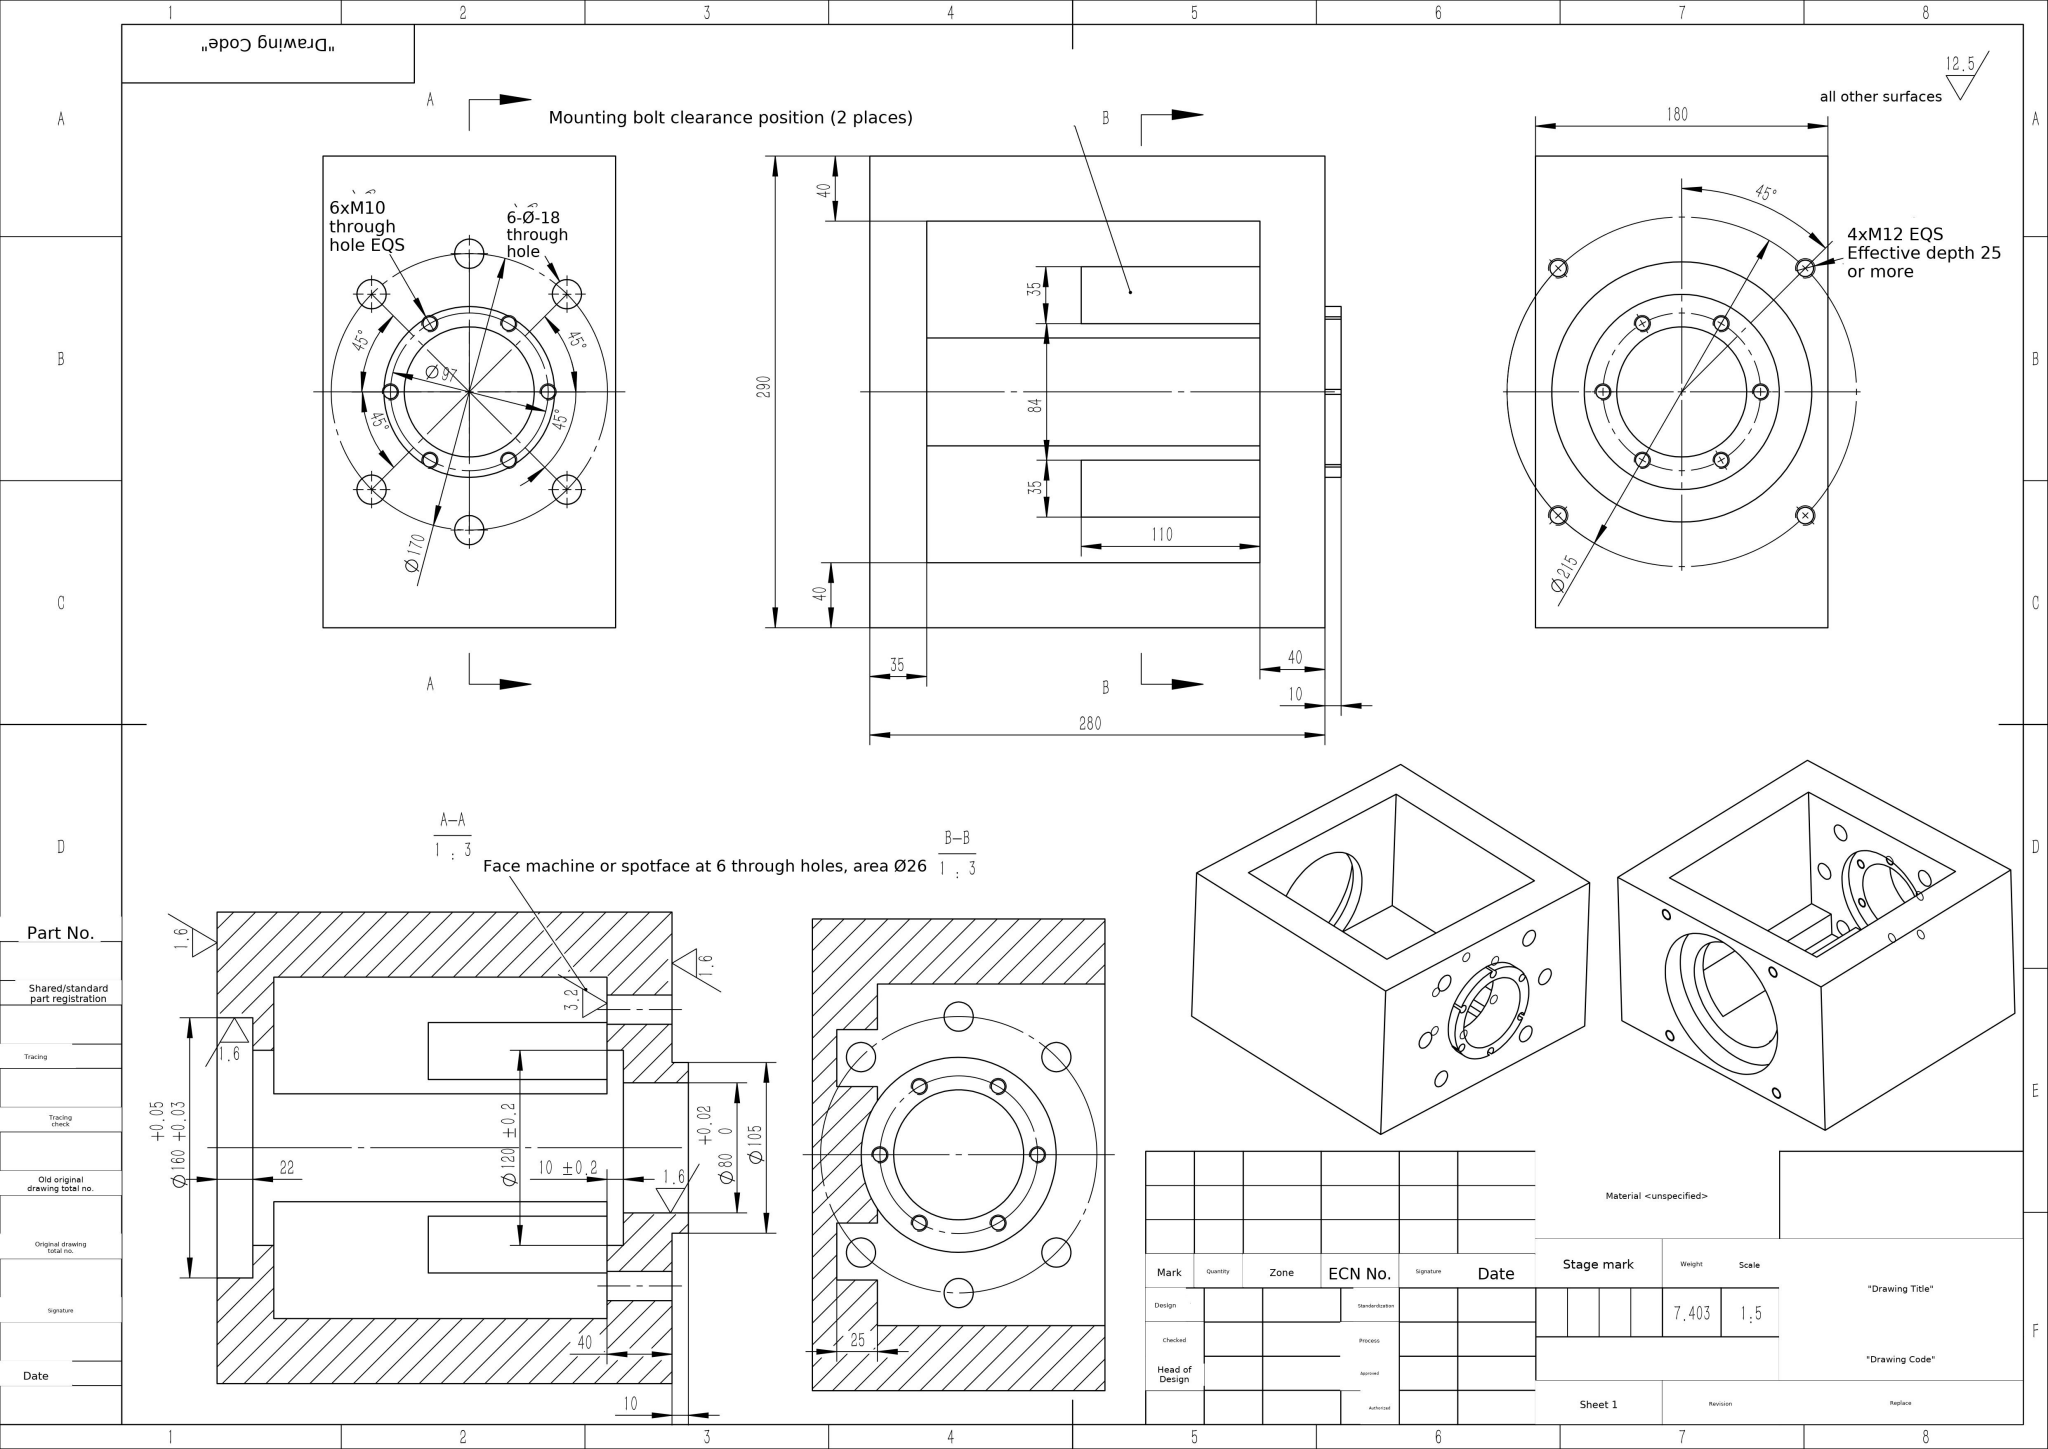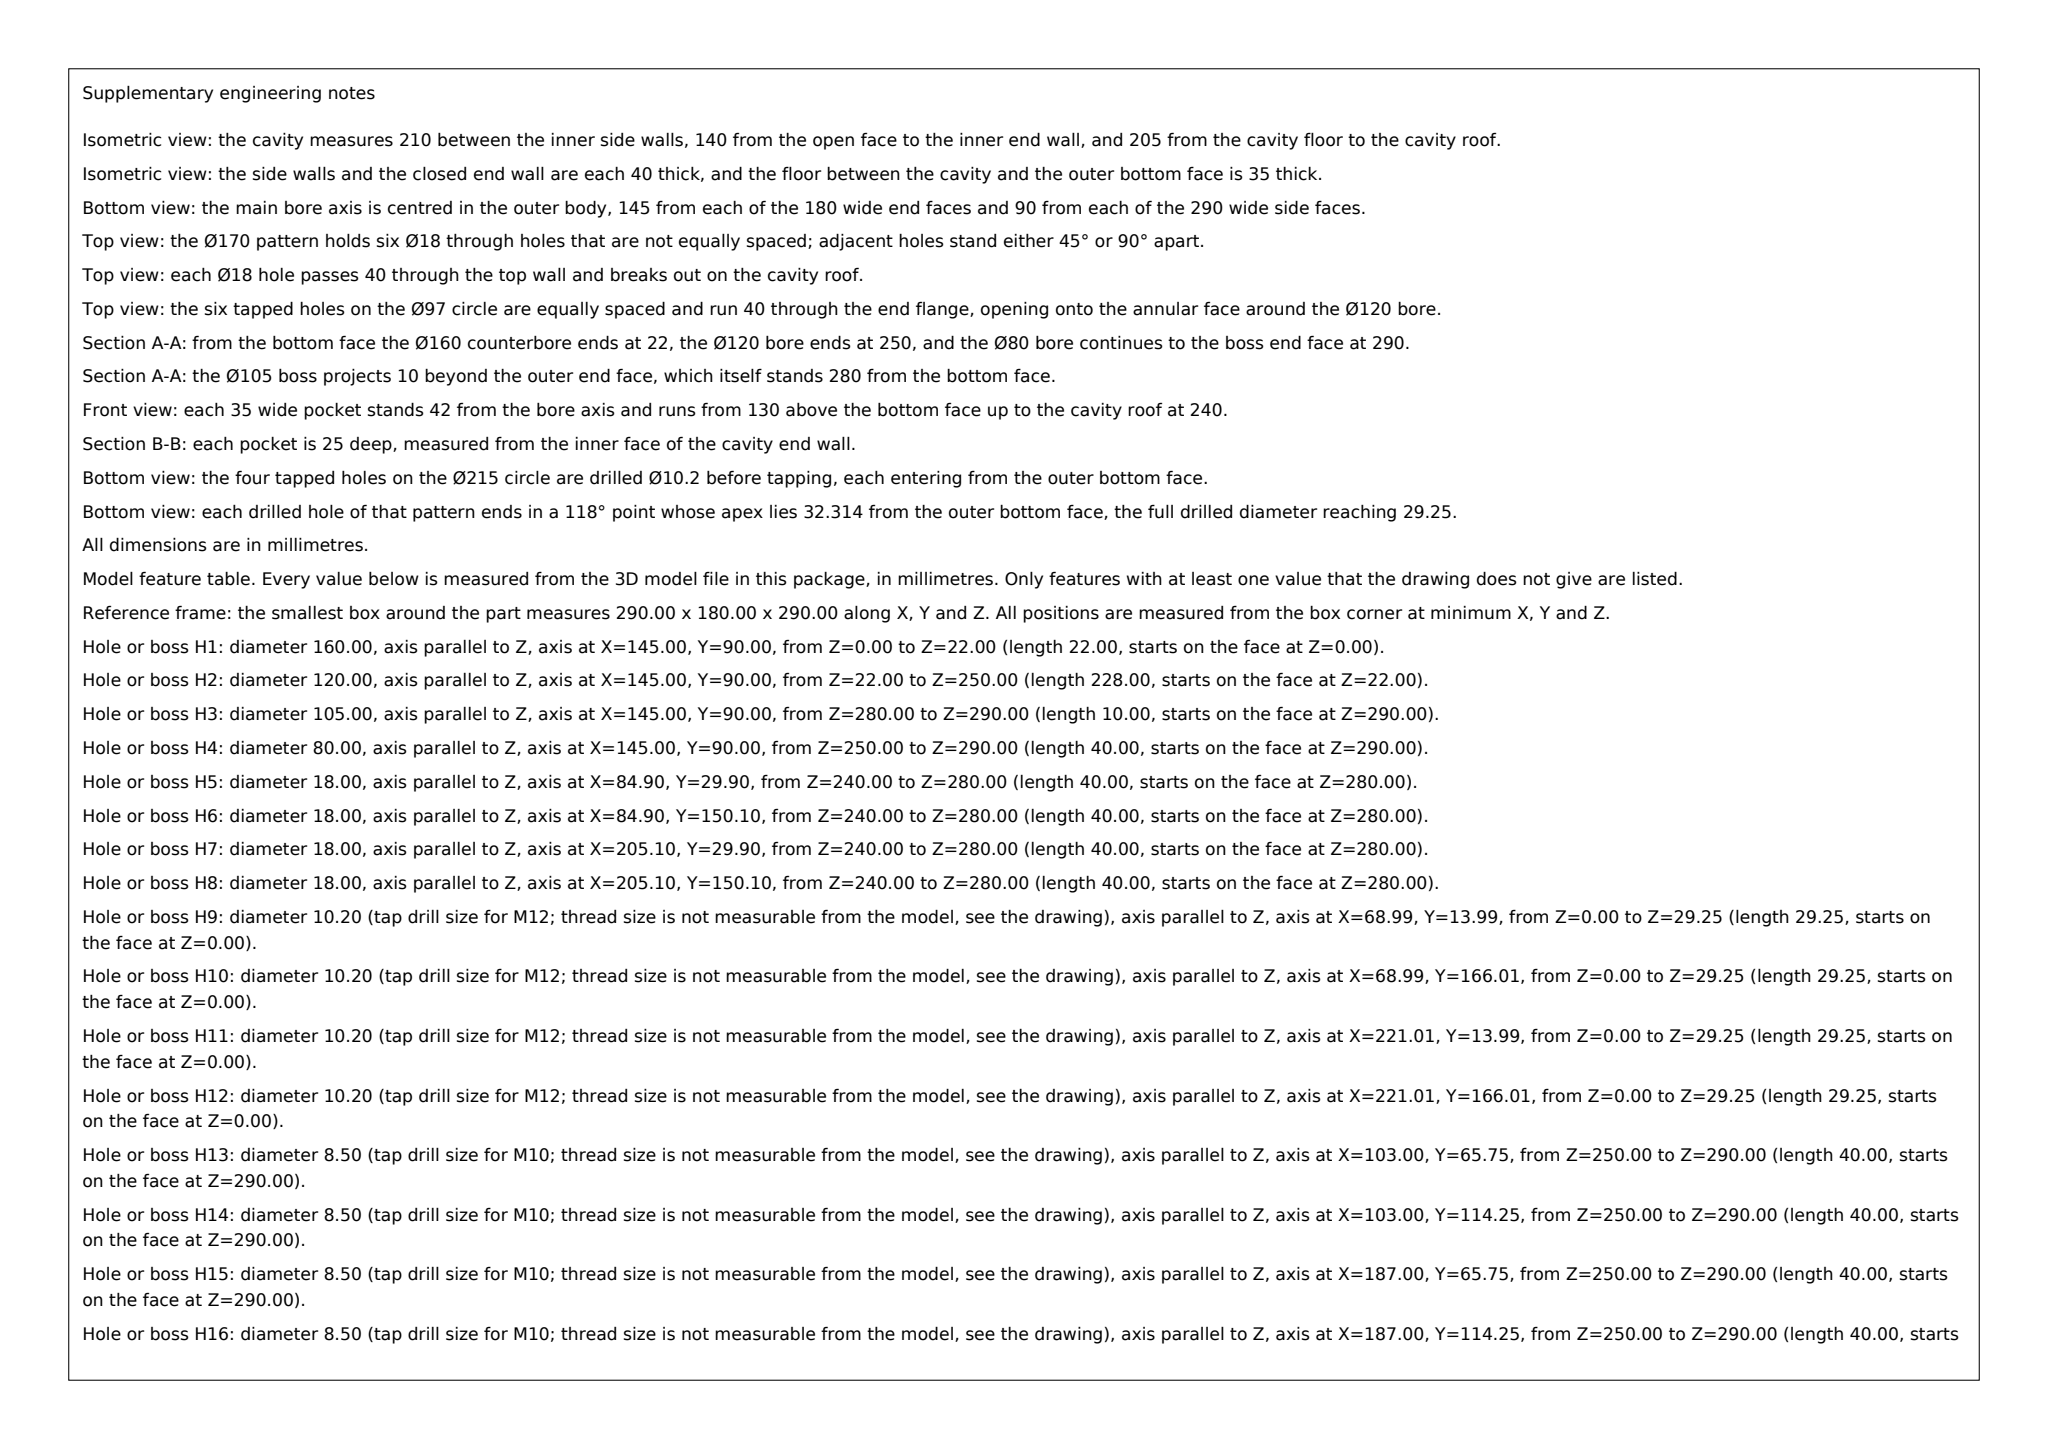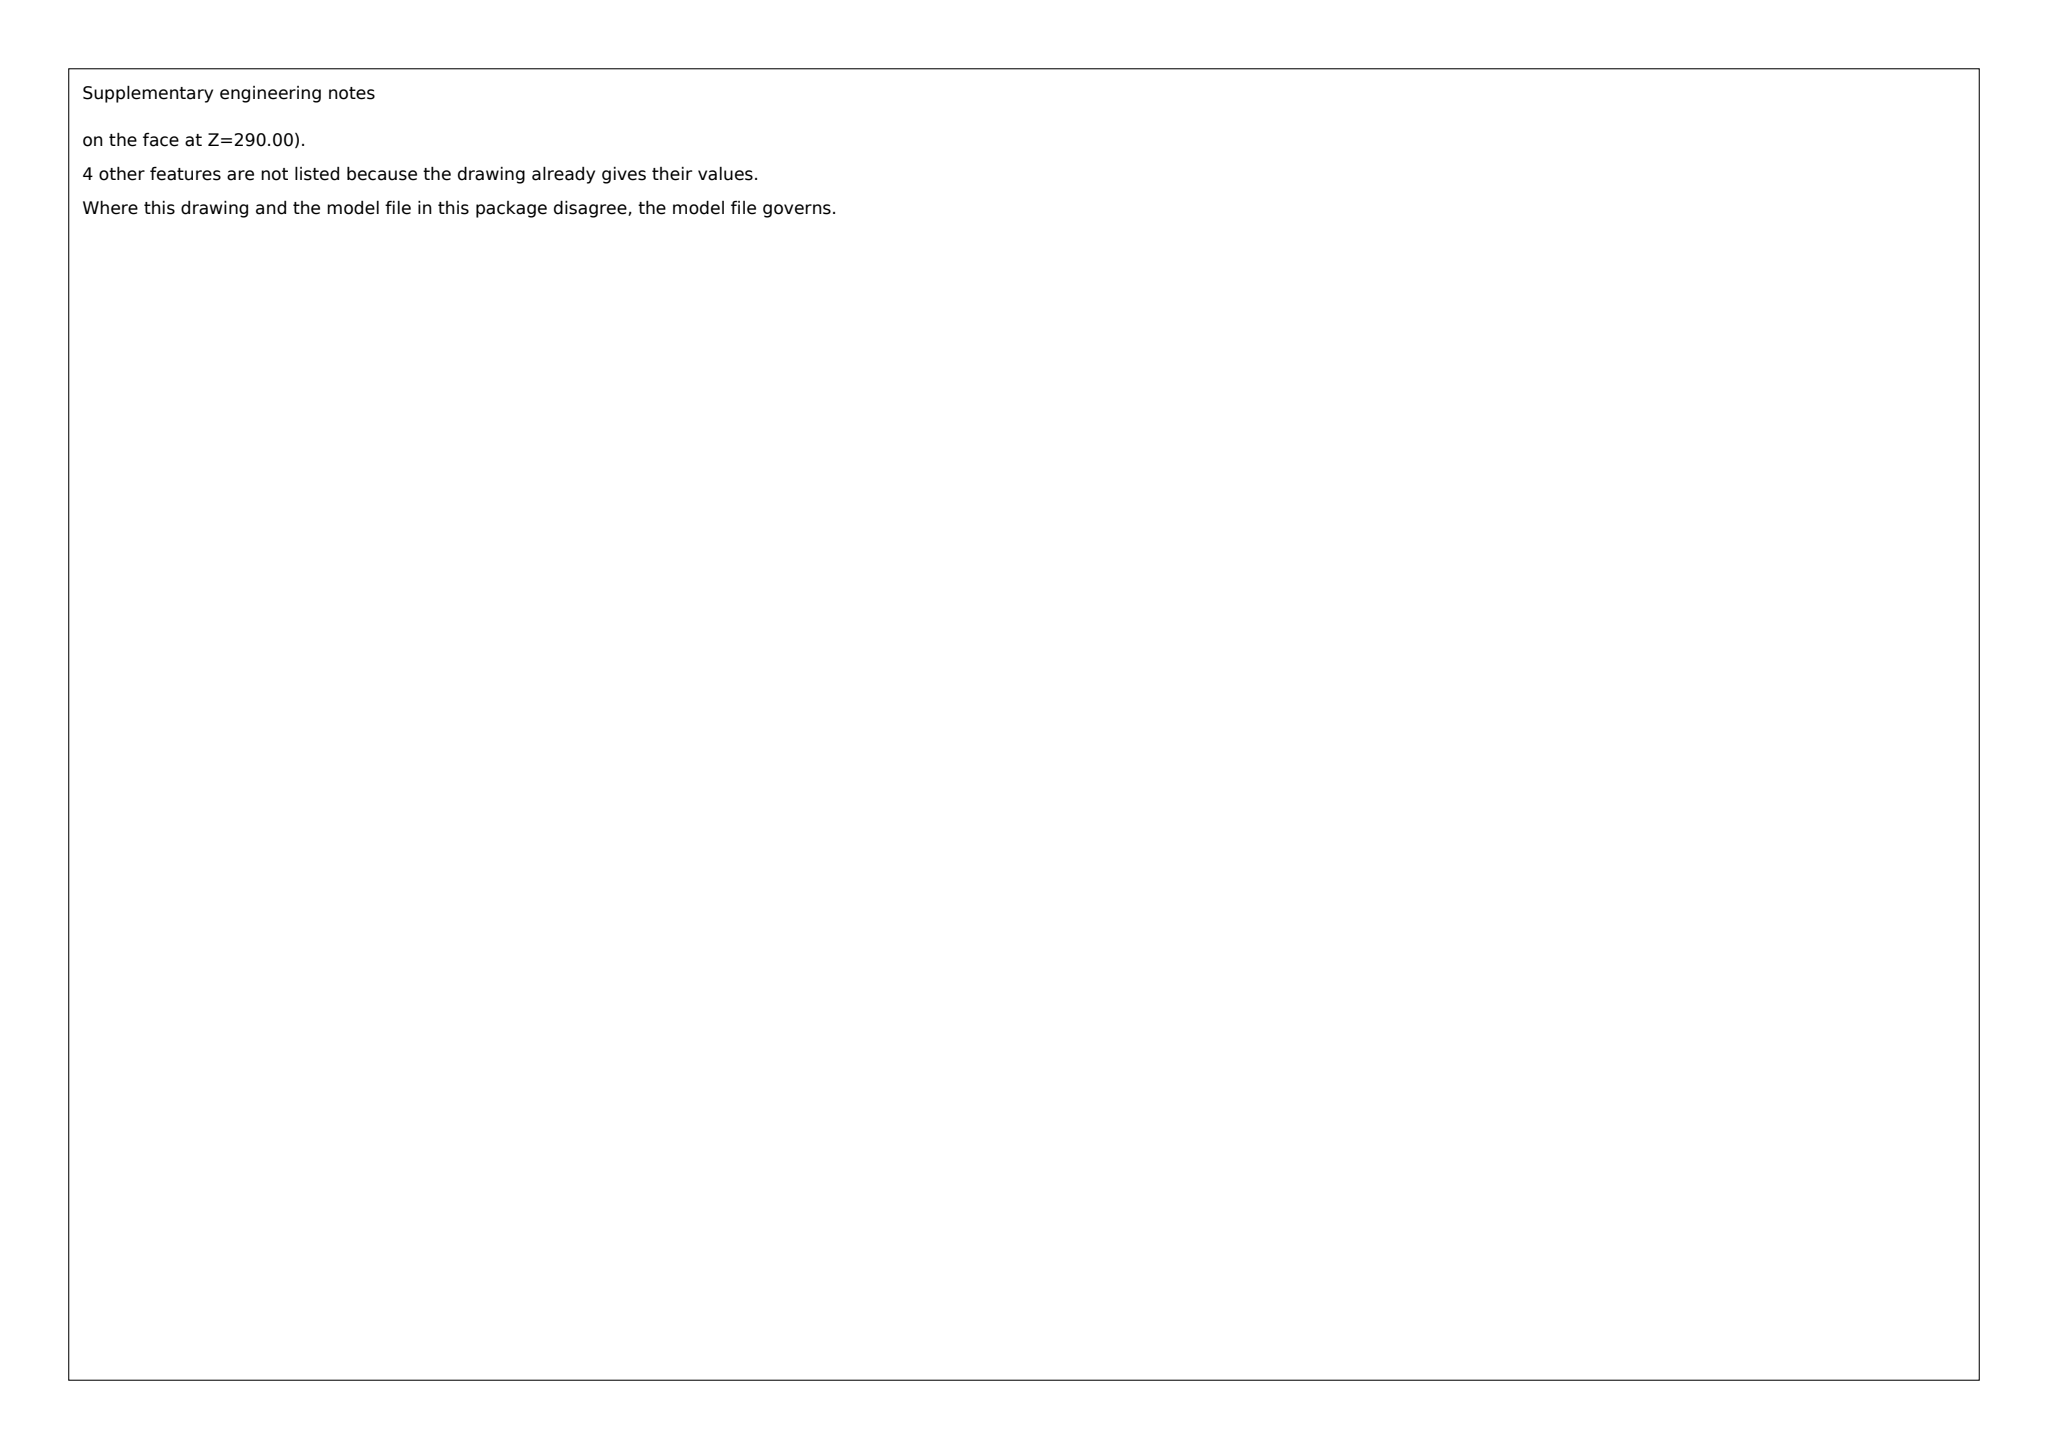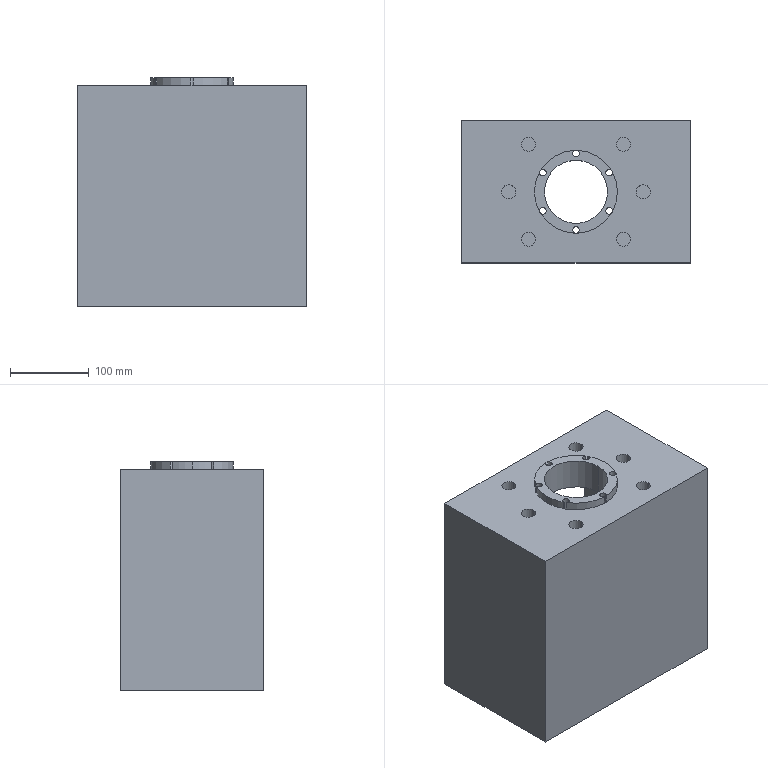Part | SolidWorks | mm | 1 solid | 77 faces | box 290 x 180 x 290 mm | volume 7402731 mm3 | cylinder 46 | plane 23 | cone 8 | commonest cylinder face diameters 8.5 x12 18 x12 10.2 x8 105 x7 120 x3 160 x2 80 x2
Drawing notes:
RECESS AT 2 LOWER Ø18 HOLES: 35 WIDE x 25 DP, FLOOR 15 FROM BASE | from the solid: y-planes 15 (x2) and 40 (x2): pocket floor at y=15, cavity floor y=40 -> 25 deep; x-planes 68/103 and 187/222 give 35 wide, bracketing Ø18 holes at x=84.9 / 205.1, y=29.9 (Ø170 PCD); outer base face y=0